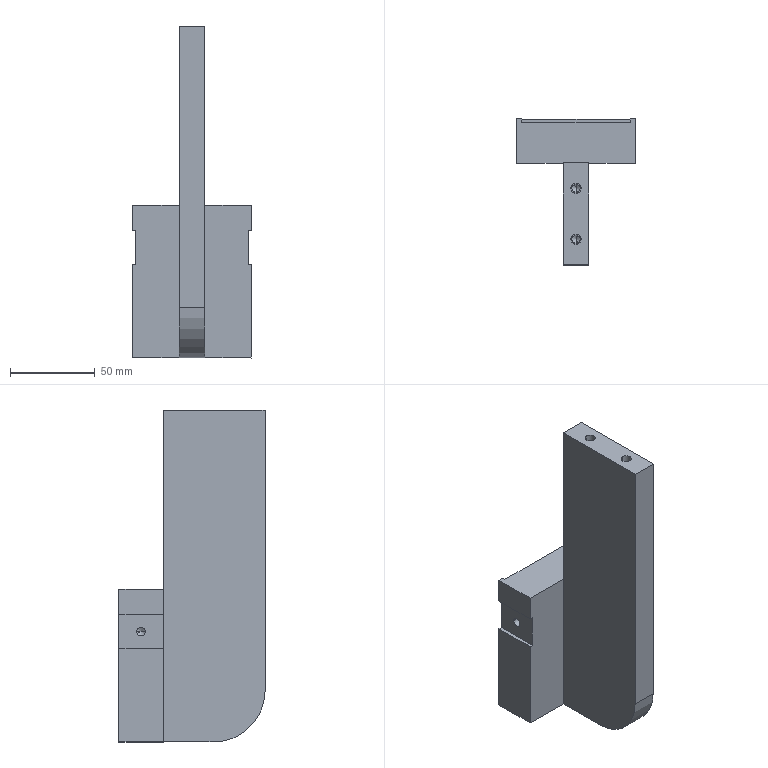Component | SolidWorks | 2SZT-2-005-1 | 1 solid | 83 faces | box 70 x 86 x 195.5 mm | volume 316947 mm3 | cylinder 33 | plane 30 | cone 20 | commonest cylinder face diameters 5 x12 6.01 x4 11 x4 6.6 x4 4.2 x4 6 x4 60 x1
build123d program:
from build123d import *

# Parameters (mm, degrees)
SKETCH1_W                                            = 195.5
SKETCH1_H                                            = 60
BOSS_EXTRUDE1_DEPTH                                  = 15
M6_TAPPED_HOLE1_D                                    = 5
M6_TAPPED_HOLE1_DEPTH                                = 15
M6_TAPPED_HOLE1_CBORE_D                              = 6
M6_TAPPED_HOLE1_CBORE_DEPTH                          = 12
M6_TAPPED_HOLE1_TIP                                  = 1.502
M6_TAPPED_HOLE2_D                                    = 5
M6_TAPPED_HOLE2_DEPTH                                = 15
M6_TAPPED_HOLE2_CBORE_D                              = 6
M6_TAPPED_HOLE2_CBORE_DEPTH                          = 12
M6_TAPPED_HOLE2_TIP                                  = 1.502
FILLET1_R                                            = 30
SKETCH11_W                                           = 70
SKETCH11_H                                           = 90
BOSS_EXTRUDE2_DEPTH                                  = 26
SKETCH12_W                                           = 64
SKETCH12_H                                           = 124.784
CUT_EXTRUDE2_DEPTH                                   = 2
M5_TAPPED_HOLE1_D                                    = 4.2
M5_TAPPED_HOLE1_DEPTH                                = 12.4
M5_TAPPED_HOLE1_CBORE_D                              = 5
M5_TAPPED_HOLE1_CBORE_DEPTH                          = 10
M5_TAPPED_HOLE1_TIP                                  = 1.262
SKETCH23_W                                           = 23.863
SKETCH23_H                                           = 20.05
SKETCH23_W_2                                         = 17.544
CUT_EXTRUDE5_DEPTH                                   = 356.964
HOLE_SIZE_ACCORDING_TO_THE_TYPE_OF_HEXAG_D           = 6.6
HOLE_SIZE_ACCORDING_TO_THE_TYPE_OF_HEXAG_DEPTH       = 30
HOLE_SIZE_ACCORDING_TO_THE_TYPE_OF_HEXAG_CBORE_D     = 11
HOLE_SIZE_ACCORDING_TO_THE_TYPE_OF_HEXAG_CBORE_DEPTH = 6.8
HOLE_SIZE_ACCORDING_TO_THE_TYPE_OF_HEXAG_TIP         = 1.983
F_6_0_6_DIAMETER_HOLE1_D                             = 6.01
F_6_0_6_DIAMETER_HOLE1_DEPTH                         = 30
F_6_0_6_DIAMETER_HOLE1_TIP                           = 1.806
M6_TAPPED_HOLE5_D                                    = 5
M6_TAPPED_HOLE5_DEPTH                                = 15
M6_TAPPED_HOLE5_TIP                                  = 1.502
M6_TAPPED_HOLE6_D                                    = 5
M6_TAPPED_HOLE6_DEPTH                                = 15
M6_TAPPED_HOLE6_TIP                                  = 1.502


with BuildPart() as part:
    # Sketch1 → Boss-Extrude1 (new body)
    with BuildSketch(Plane(origin=(-186.7, 0, 0), x_dir=(0, -1, 0), z_dir=(-1, 0, 0))):
        with Locations((-180.15, -148.03)):
            Rectangle(SKETCH1_W, SKETCH1_H)
    extrude(amount=-BOSS_EXTRUDE1_DEPTH)

    # M6 Tapped Hole1
    with Locations(Plane.XZ.offset(-82.4)):
        with Locations((-179.2, -133.03)):
            CounterBoreHole(M6_TAPPED_HOLE1_D / 2, M6_TAPPED_HOLE1_CBORE_D / 2, M6_TAPPED_HOLE1_CBORE_DEPTH, depth=M6_TAPPED_HOLE1_DEPTH)
            with Locations((0, 0, -(M6_TAPPED_HOLE1_DEPTH + M6_TAPPED_HOLE1_TIP / 2))):  # 118° drill point
                Cone(0, M6_TAPPED_HOLE1_D / 2, M6_TAPPED_HOLE1_TIP, mode=Mode.SUBTRACT)

    # M6 Tapped Hole2
    with Locations(Plane.XZ.offset(-82.4)):
        with Locations((-179.2, -163.03)):
            CounterBoreHole(M6_TAPPED_HOLE2_D / 2, M6_TAPPED_HOLE2_CBORE_D / 2, M6_TAPPED_HOLE2_CBORE_DEPTH, depth=M6_TAPPED_HOLE2_DEPTH)
            with Locations((0, 0, -(M6_TAPPED_HOLE2_DEPTH + M6_TAPPED_HOLE2_TIP / 2))):  # 118° drill point
                Cone(0, M6_TAPPED_HOLE2_D / 2, M6_TAPPED_HOLE2_TIP, mode=Mode.SUBTRACT)

    # Fillet1
    fillet1_edges = [part.edges().sort_by_distance(p)[0] for p in [
        (-179.2, 277.9, -178.03),
    ]]
    fillet(fillet1_edges, radius=FILLET1_R)

    # Sketch11 → Boss-Extrude2 (add)
    with BuildSketch(Plane.XY.offset(-118.03)):
        with Locations((-179.2, 232.9)):
            Rectangle(SKETCH11_W, SKETCH11_H)
    extrude(amount=BOSS_EXTRUDE2_DEPTH)

    # Sketch12 → Cut-Extrude2 (cut)
    with BuildSketch(Plane.XY.offset(-92.03)):
        with Locations((-179.2, 213.508)):
            Rectangle(SKETCH12_W, SKETCH12_H)
    extrude(amount=-CUT_EXTRUDE2_DEPTH, mode=Mode.SUBTRACT)

    # M5 Tapped Hole1
    with Locations(Plane.XY.offset(-94.03)):
        with Locations((-179.2, 245.9), (-179.2, 215.9)):
            CounterBoreHole(M5_TAPPED_HOLE1_D / 2, M5_TAPPED_HOLE1_CBORE_D / 2, M5_TAPPED_HOLE1_CBORE_DEPTH, depth=M5_TAPPED_HOLE1_DEPTH)
            with Locations((0, 0, -(M5_TAPPED_HOLE1_DEPTH + M5_TAPPED_HOLE1_TIP / 2))):  # 118° drill point
                Cone(0, M5_TAPPED_HOLE1_D / 2, M5_TAPPED_HOLE1_TIP, mode=Mode.SUBTRACT)

    # Sketch23 → Cut-Extrude5 (cut, through all)
    with BuildSketch(Plane(origin=(0, 0, -118.03), x_dir=(-1, 0, 0), z_dir=(0, 0, -1))):
        with Locations((134.268, 212.9)):
            Rectangle(SKETCH23_W, SKETCH23_H)
        with Locations((220.972, 212.9)):
            Rectangle(SKETCH23_W_2, SKETCH23_H)
    extrude(amount=-CUT_EXTRUDE5_DEPTH, mode=Mode.SUBTRACT)

    # Hole Size according to the type of hexag
    with Locations(Plane.XY.offset(-94.03)):
        with Locations((-179.2, 267.9), (-179.2, 229.9)):
            CounterBoreHole(HOLE_SIZE_ACCORDING_TO_THE_TYPE_OF_HEXAG_D / 2, HOLE_SIZE_ACCORDING_TO_THE_TYPE_OF_HEXAG_CBORE_D / 2, HOLE_SIZE_ACCORDING_TO_THE_TYPE_OF_HEXAG_CBORE_DEPTH, depth=HOLE_SIZE_ACCORDING_TO_THE_TYPE_OF_HEXAG_DEPTH)
            with Locations((0, 0, -(HOLE_SIZE_ACCORDING_TO_THE_TYPE_OF_HEXAG_DEPTH + HOLE_SIZE_ACCORDING_TO_THE_TYPE_OF_HEXAG_TIP / 2))):  # 118° drill point
                Cone(0, HOLE_SIZE_ACCORDING_TO_THE_TYPE_OF_HEXAG_D / 2, HOLE_SIZE_ACCORDING_TO_THE_TYPE_OF_HEXAG_TIP, mode=Mode.SUBTRACT)

    # 6.0 _6_ Diameter Hole1
    with Locations(Plane.XY.offset(-94.03)):
        with Locations((-179.2, 255.9), (-179.2, 197.9)):
            Hole(F_6_0_6_DIAMETER_HOLE1_D / 2, depth=F_6_0_6_DIAMETER_HOLE1_DEPTH)
            with Locations((0, 0, -(F_6_0_6_DIAMETER_HOLE1_DEPTH + F_6_0_6_DIAMETER_HOLE1_TIP / 2))):  # 118° drill point
                Cone(0, F_6_0_6_DIAMETER_HOLE1_D / 2, F_6_0_6_DIAMETER_HOLE1_TIP, mode=Mode.SUBTRACT)

    # M6 Tapped Hole5
    with Locations(Plane(origin=(-146.2, 0, 0), x_dir=(0, 0, -1), z_dir=(1, 0, 0))):
        with Locations((105.03, 212.9)):
            Hole(M6_TAPPED_HOLE5_D / 2, depth=M6_TAPPED_HOLE5_DEPTH)
            with Locations((0, 0, -(M6_TAPPED_HOLE5_DEPTH + M6_TAPPED_HOLE5_TIP / 2))):  # 118° drill point
                Cone(0, M6_TAPPED_HOLE5_D / 2, M6_TAPPED_HOLE5_TIP, mode=Mode.SUBTRACT)

    # M6 Tapped Hole6
    with Locations(Plane.ZY.offset(212.2)):
        with Locations((-105.03, 212.9)):
            Hole(M6_TAPPED_HOLE6_D / 2, depth=M6_TAPPED_HOLE6_DEPTH)
            with Locations((0, 0, -(M6_TAPPED_HOLE6_DEPTH + M6_TAPPED_HOLE6_TIP / 2))):  # 118° drill point
                Cone(0, M6_TAPPED_HOLE6_D / 2, M6_TAPPED_HOLE6_TIP, mode=Mode.SUBTRACT)


solid = part.part

# Placed as in the assembly
solid = solid.moved(Location((1134.464, 466.123, -170.296), (-90, 0, 0)))